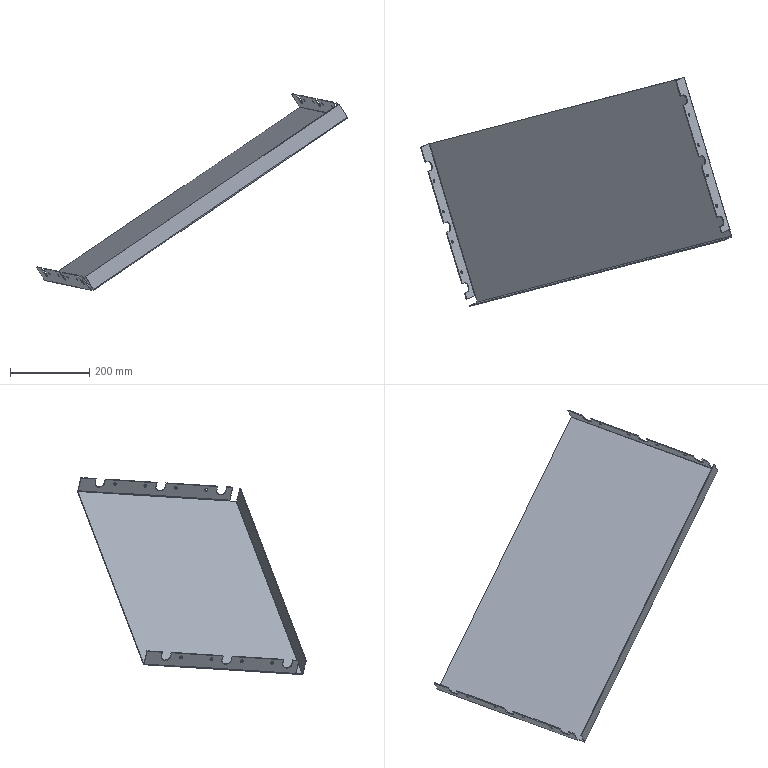Component | SolidWorks | CrusherFrameSideCover-1 | 1 solid | 78 faces | volume 786084 mm3 | plane 44 | cylinder 34 | commonest cylinder face diameters 7 x16 24 x12 6 x3 2 x3